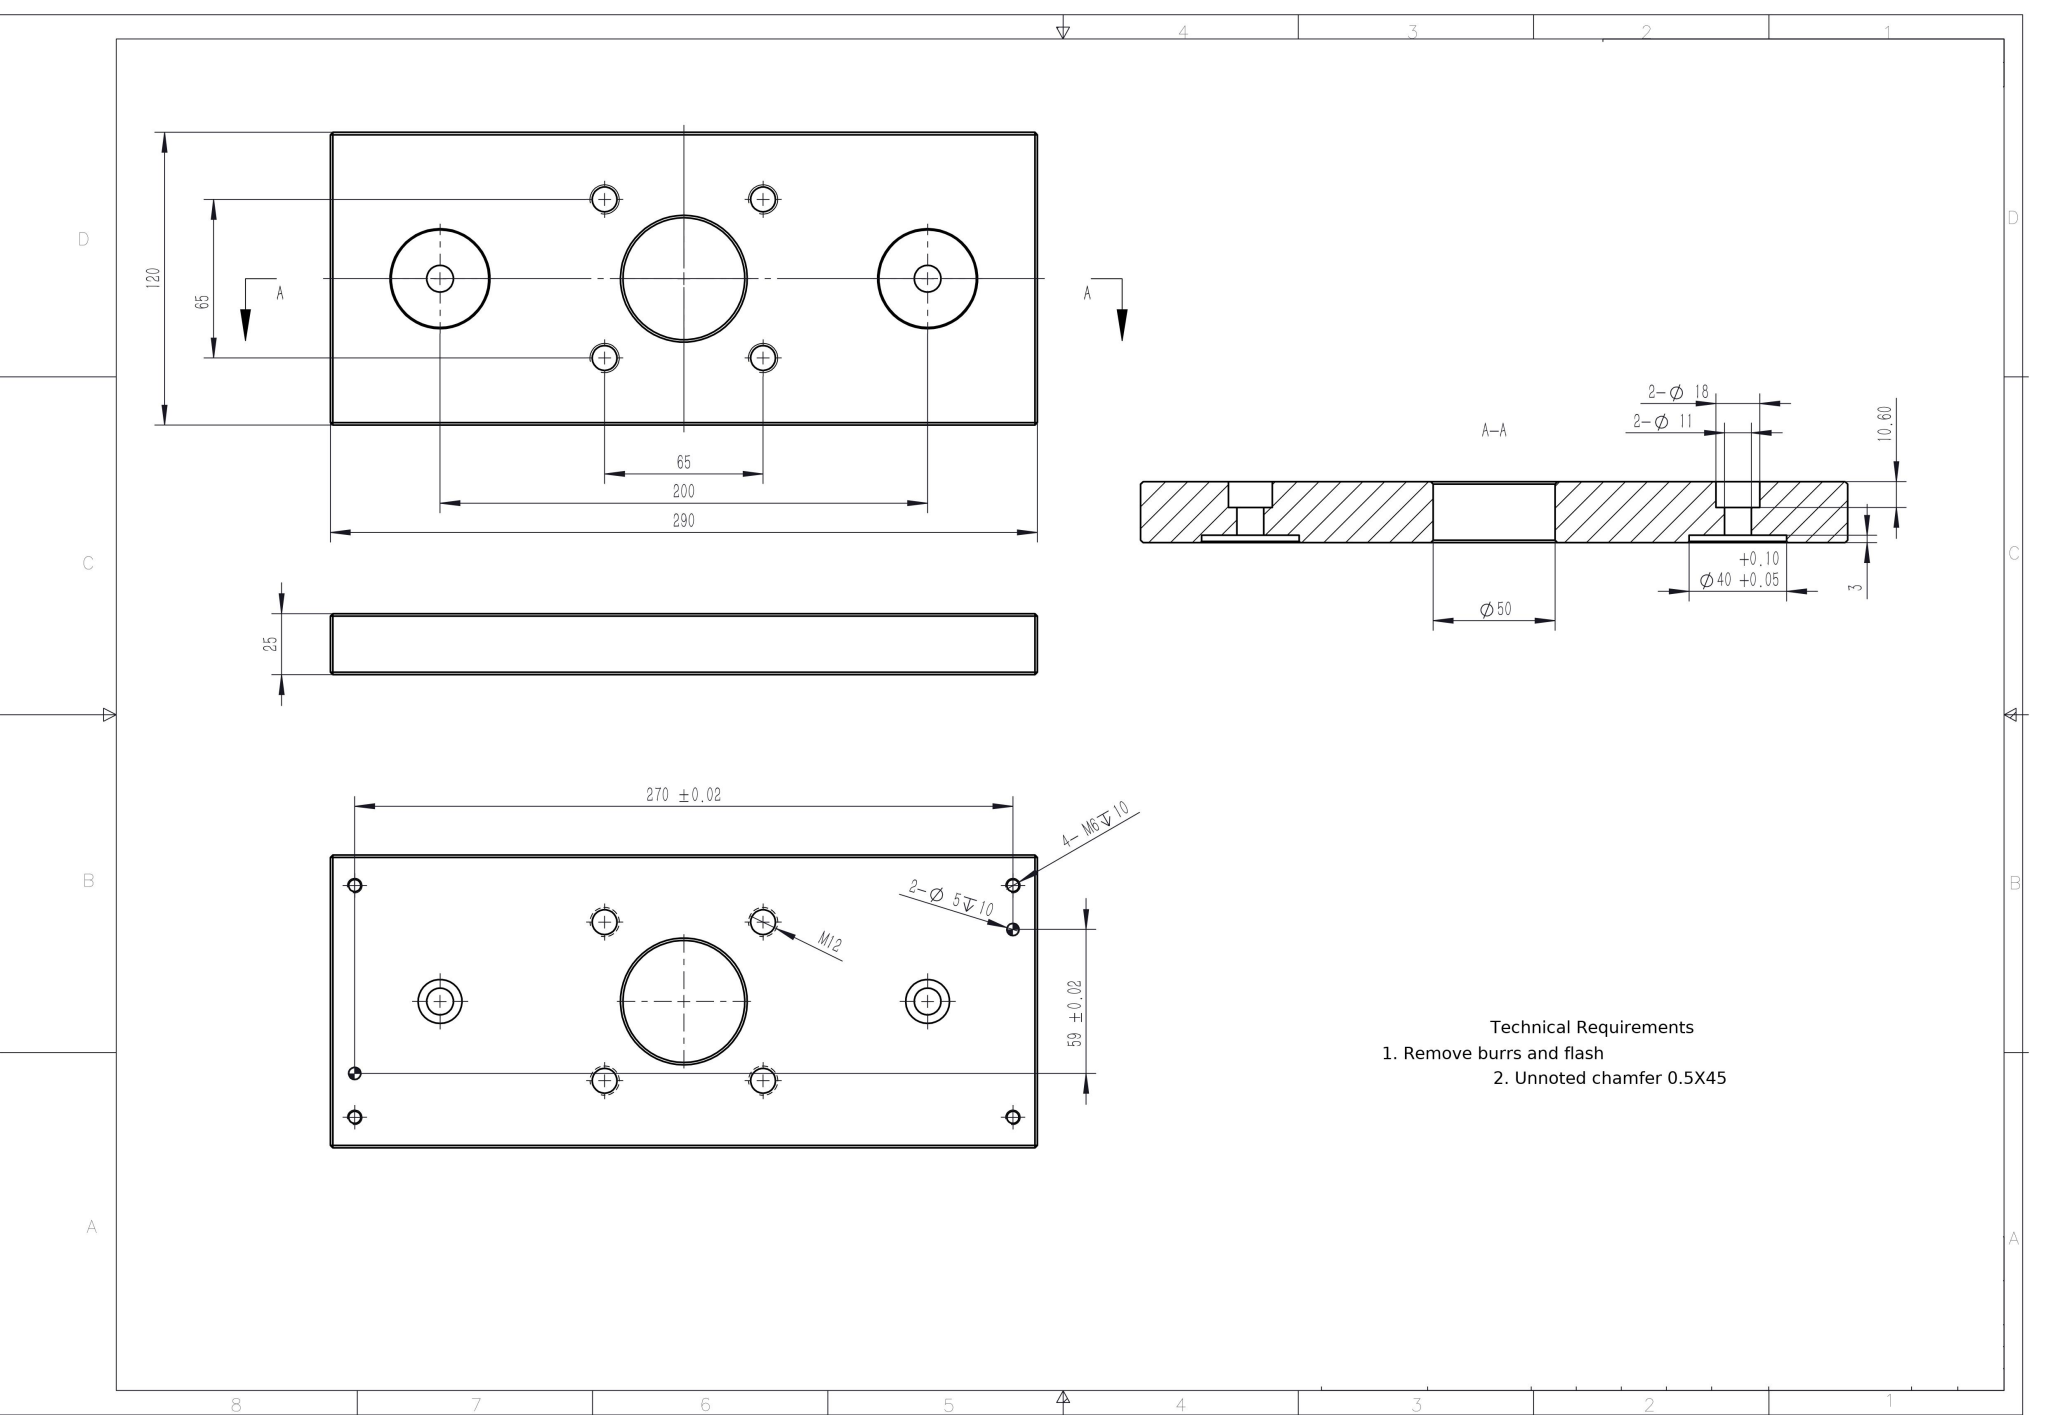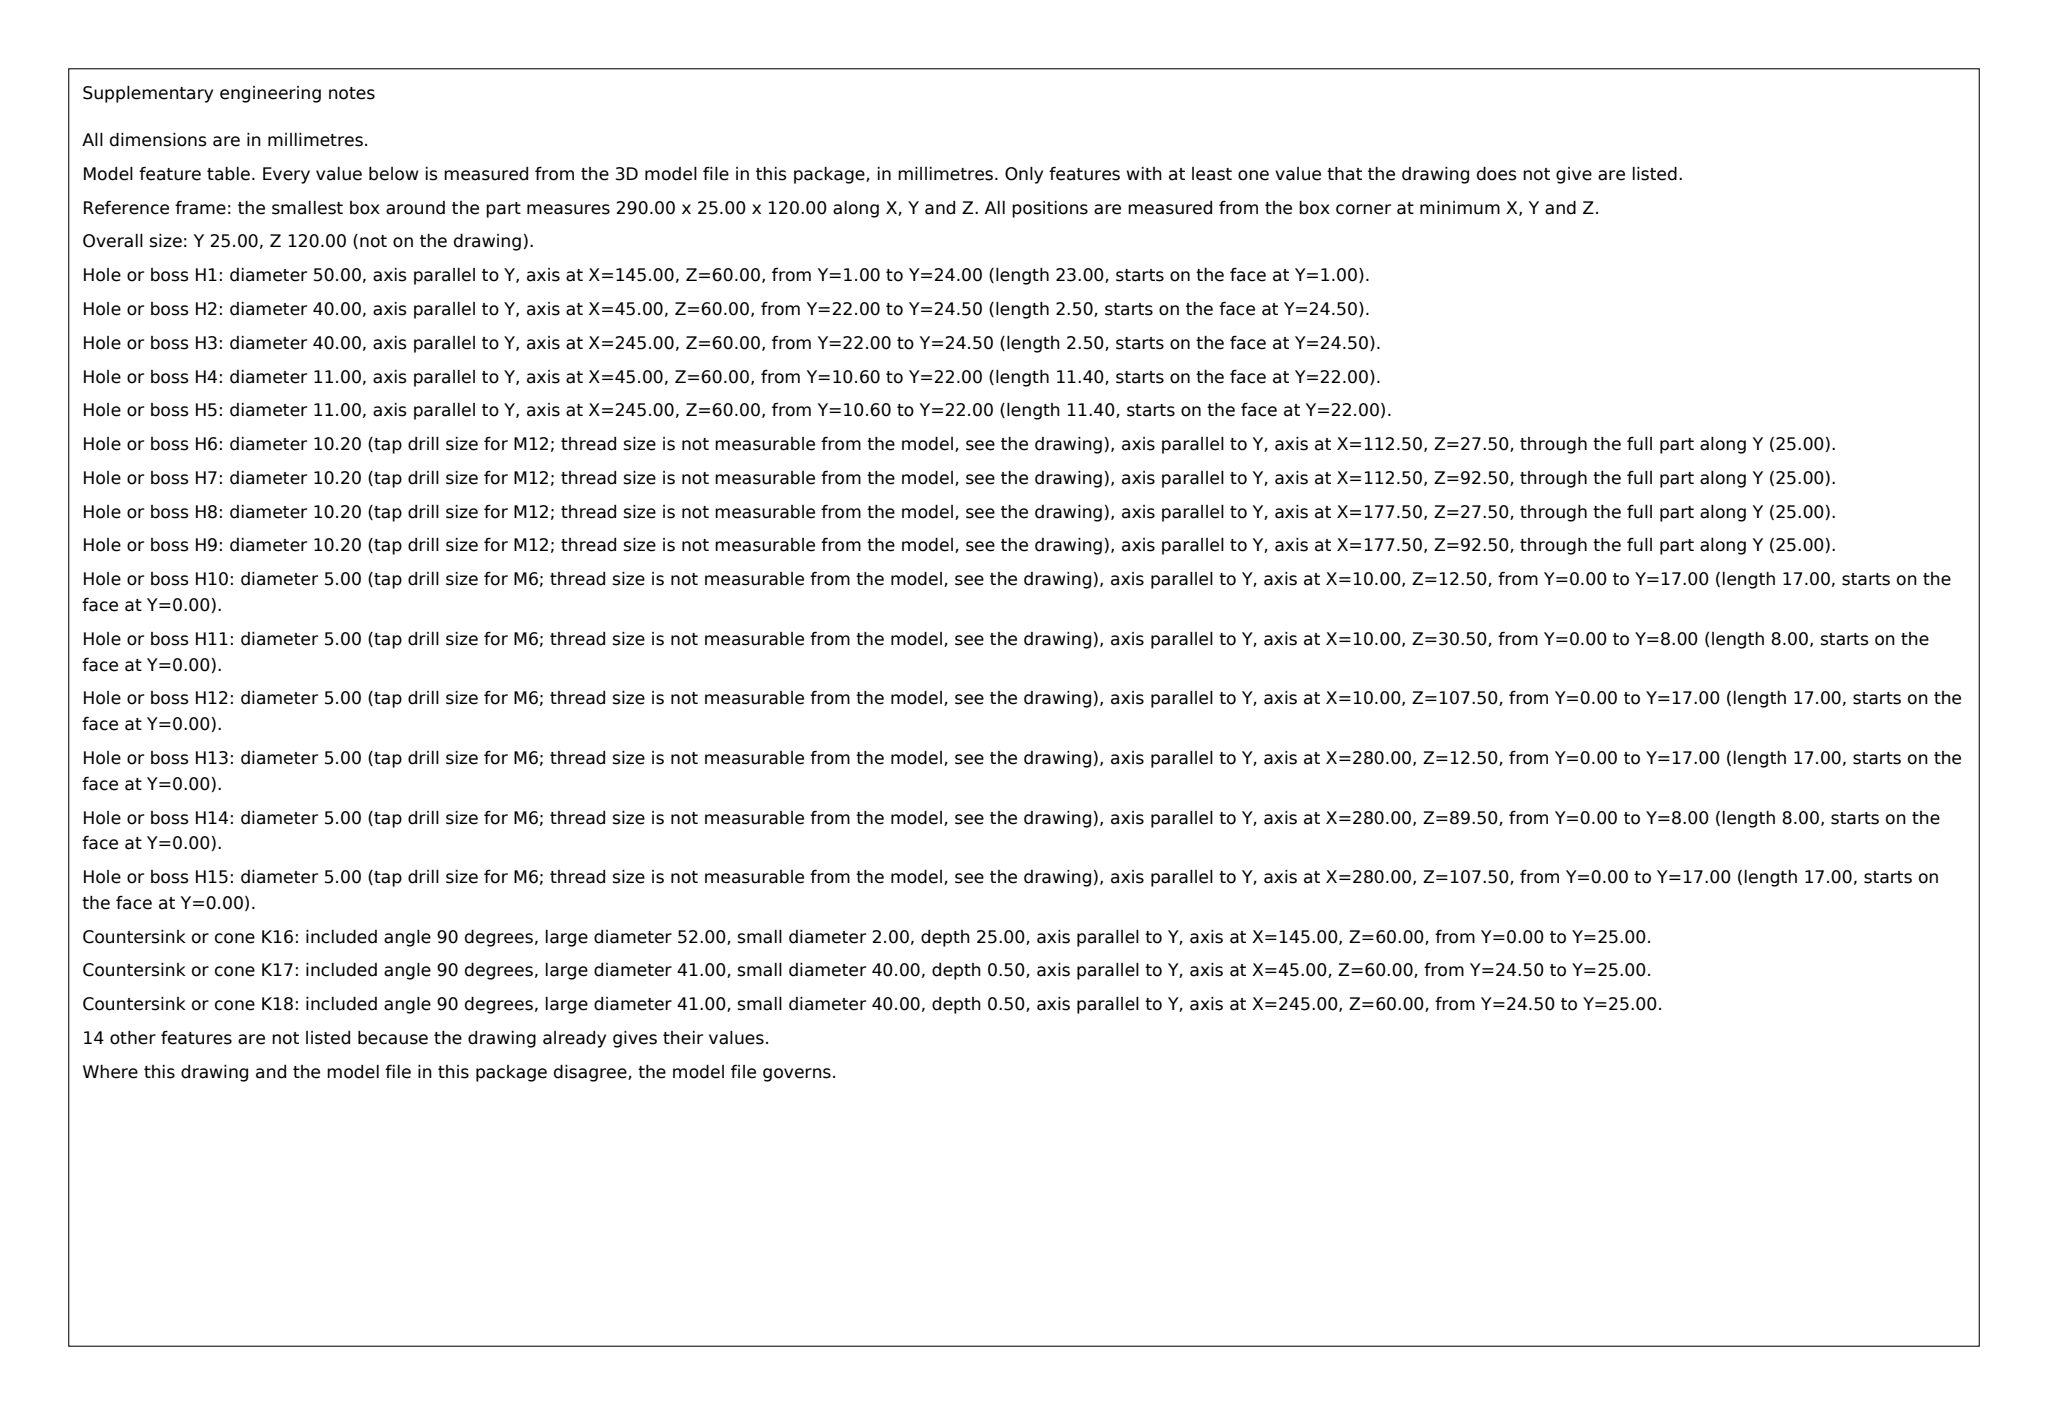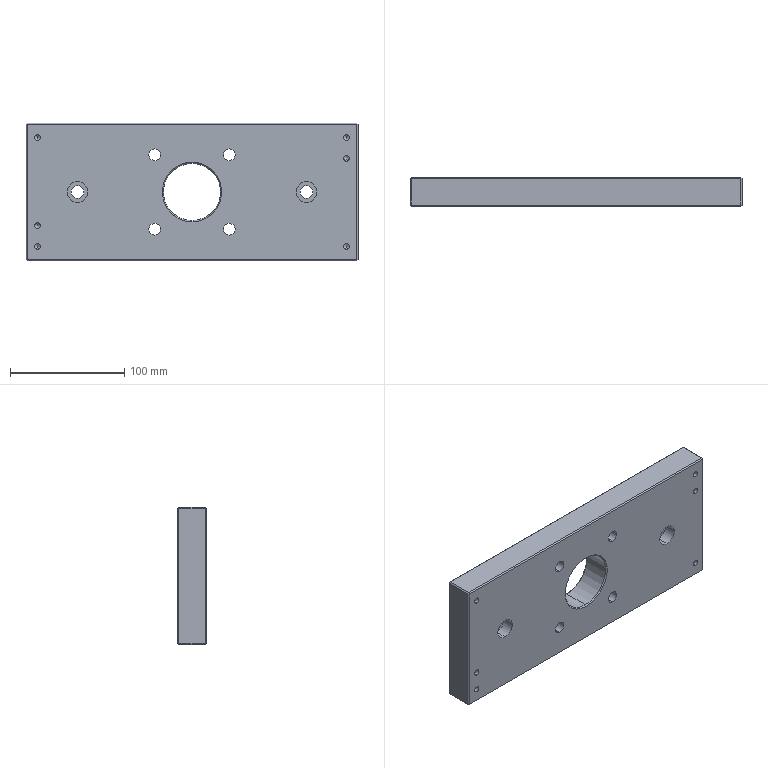Part | SolidWorks | mm | 1 solid | 84 faces | box 290 x 25 x 120 mm | volume 794876 mm3 | cylinder 34 | plane 30 | cone 20 | commonest cylinder face diameters 5 x12 10.2 x8 40 x4 18 x4 11 x4 50 x2
build123d program:
from build123d import *

# Parameters (mm, degrees)
SKETCH1_W                                        = 290
SKETCH1_H                                        = 120
BOSS_EXTRUDE1_DEPTH                              = 25
F_12_0_12_DIAMETER_HOLE2_D                       = 50
M12_TAPPED_HOLE1_D                               = 10.2
M12_TAPPED_HOLE1_DEPTH                           = 32.75
M12_TAPPED_HOLE1_TIP                             = 3.064
M10_HEX_SOCKET_HEAD_CAP_SCREW_CBORE1_D           = 11
M10_HEX_SOCKET_HEAD_CAP_SCREW_CBORE1_CBORE_D     = 18
M10_HEX_SOCKET_HEAD_CAP_SCREW_CBORE1_CBORE_DEPTH = 10.6
SKETCH10_R                                       = 20
CUT_EXTRUDE1_DEPTH                               = 3
CHAMFER1_SIZE                                    = 0.5
CHAMFER2_SIZE                                    = 1
M6_TAPPED_HOLE1_D                                = 5
M6_TAPPED_HOLE1_DEPTH                            = 17
M6_TAPPED_HOLE1_TIP                              = 1.502
SIZE_MM_DOWEL_PIN_HOLE1_D                        = 5
SIZE_MM_DOWEL_PIN_HOLE1_DEPTH                    = 8
SIZE_MM_DOWEL_PIN_HOLE1_TIP                      = 1.502


with BuildPart() as part:
    # Sketch1 → Boss-Extrude1 (new body)
    with BuildSketch(Plane(origin=(0, 0, 0), x_dir=(1, 0, 0), z_dir=(0, 1, 0))):
        Rectangle(SKETCH1_W, SKETCH1_H)
    extrude(amount=BOSS_EXTRUDE1_DEPTH)

    # 12.0 _12_ Diameter Hole2 (through all)
    with Locations(Plane(origin=(0, 25, 0), x_dir=(1, 0, 0), z_dir=(0, 1, 0))):
        with Locations((0, 0)):
            Hole(F_12_0_12_DIAMETER_HOLE2_D / 2)

    # M12 Tapped Hole1
    with Locations(Plane(origin=(0, 25, 0), x_dir=(1, 0, 0), z_dir=(0, 1, 0))):
        with Locations((-32.5, 32.5), (32.5, 32.5), (-32.5, -32.5), (32.5, -32.5)):
            Hole(M12_TAPPED_HOLE1_D / 2, depth=M12_TAPPED_HOLE1_DEPTH)
            with Locations((0, 0, -(M12_TAPPED_HOLE1_DEPTH + M12_TAPPED_HOLE1_TIP / 2))):  # 118° drill point
                Cone(0, M12_TAPPED_HOLE1_D / 2, M12_TAPPED_HOLE1_TIP, mode=Mode.SUBTRACT)

    # M10 Hex Socket Head Cap Screw CBORE1 (through all)
    with Locations(Plane(origin=(0, 0, 0), x_dir=(-1, 0, 0), z_dir=(0, -1, 0))):
        with Locations((-100, 0), (100, 0)):
            CounterBoreHole(M10_HEX_SOCKET_HEAD_CAP_SCREW_CBORE1_D / 2, M10_HEX_SOCKET_HEAD_CAP_SCREW_CBORE1_CBORE_D / 2, M10_HEX_SOCKET_HEAD_CAP_SCREW_CBORE1_CBORE_DEPTH)

    # Sketch10 → Cut-Extrude1 (cut)
    with BuildSketch(Plane(origin=(0, 25, 0), x_dir=(1, 0, 0), z_dir=(0, 1, 0))):
        with Locations(Location((-100, 0, 0), (0, 0, 270))):
            Circle(SKETCH10_R)
        with Locations(Location((100, 0, 0), (0, 0, 270))):
            Circle(SKETCH10_R)
    extrude(amount=-CUT_EXTRUDE1_DEPTH, mode=Mode.SUBTRACT)

    # Chamfer1
    chamfer1_edges = [part.edges().sort_by_distance(p)[0] for p in [
        (-100, 25, -20),
        (100, 25, -20),
    ]]
    chamfer(chamfer1_edges, length=CHAMFER1_SIZE)

    # Chamfer2
    chamfer2_edges = [part.edges().sort_by_distance(p)[0] for p in [
        (-145, 25, 0),
        (0, 25, 60),
        (25, 25, 0),
        (25, 0, 0),
        (145, 25, 0),
        (0, 0, 60),
        (-145, 0, 0),
        (0, 0, -60),
        (145, 0, 0),
        (0, 25, -60),
        (145, 12.5, 60),
        (-145, 12.5, 60),
        (-145, 12.5, -60),
        (145, 12.5, -60),
    ]]
    chamfer(chamfer2_edges, length=CHAMFER2_SIZE)

    # M6 Tapped Hole1
    with Locations(Plane(origin=(0, 0, 0), x_dir=(-1, 0, 0), z_dir=(0, -1, 0))):
        with Locations((135, -47.5), (135, 47.5), (-135, -47.5), (-135, 47.5)):
            Hole(M6_TAPPED_HOLE1_D / 2, depth=M6_TAPPED_HOLE1_DEPTH)
            with Locations((0, 0, -(M6_TAPPED_HOLE1_DEPTH + M6_TAPPED_HOLE1_TIP / 2))):  # 118° drill point
                Cone(0, M6_TAPPED_HOLE1_D / 2, M6_TAPPED_HOLE1_TIP, mode=Mode.SUBTRACT)

    # Size mm Dowel Pin Hole1
    with Locations(Plane(origin=(0, 0, 0), x_dir=(-1, 0, 0), z_dir=(0, -1, 0))):
        with Locations((135, 29.5), (-135, -29.5)):
            Hole(SIZE_MM_DOWEL_PIN_HOLE1_D / 2, depth=SIZE_MM_DOWEL_PIN_HOLE1_DEPTH)
            with Locations((0, 0, -(SIZE_MM_DOWEL_PIN_HOLE1_DEPTH + SIZE_MM_DOWEL_PIN_HOLE1_TIP / 2))):  # 118° drill point
                Cone(0, SIZE_MM_DOWEL_PIN_HOLE1_D / 2, SIZE_MM_DOWEL_PIN_HOLE1_TIP, mode=Mode.SUBTRACT)


solid = part.part